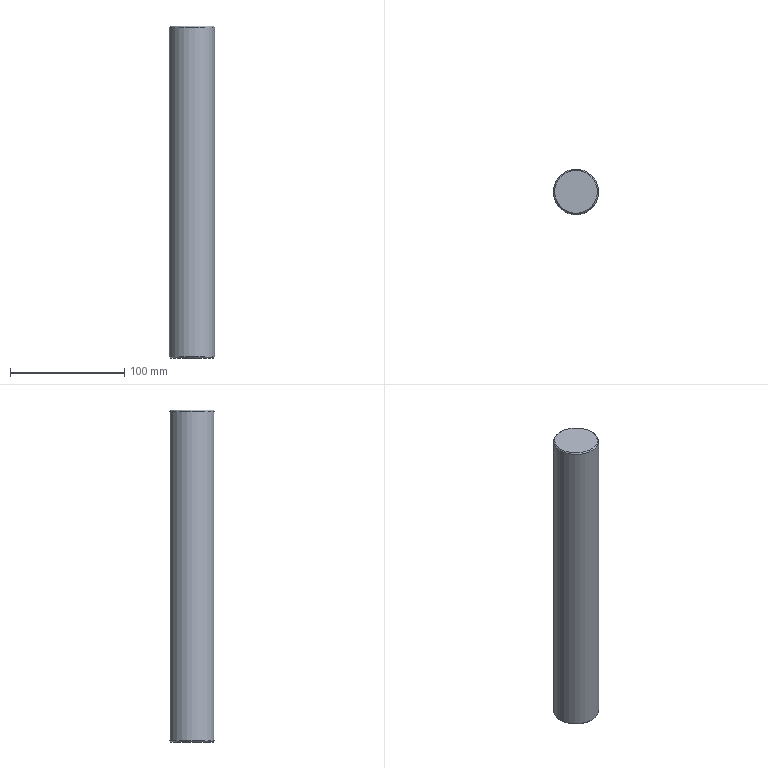Component | NX | STUD | 1 solid | 5 faces | box 39.47 x 39.47 x 290 mm | volume 354647 mm3 | plane 2 | cone 2 | cylinder 1 | commonest cylinder face diameters 39.467 x1
STEP:
#1=CARTESIAN_POINT('',(0.,0.,0.));
#2=DIRECTION('',(0.,0.,1.));
#3=DIRECTION('',(1.,0.,0.));
#4=AXIS2_PLACEMENT_3D('',#1,#2,#3);
#5=CARTESIAN_POINT('',(-41.267,165.,310.));
#6=VERTEX_POINT('',#5);
#7=CARTESIAN_POINT('',(-60.,165.,310.));
#8=DIRECTION('',(0.,0.,1.));
#9=DIRECTION('',(1.,0.,0.));
#10=AXIS2_PLACEMENT_3D('',#7,#8,#9);
#11=CIRCLE('',#10,18.733);
#12=CARTESIAN_POINT('',(-60.,165.,310.));
#13=DIRECTION('',(0.,0.,1.));
#14=DIRECTION('',(1.,0.,0.));
#15=AXIS2_PLACEMENT_3D('',#12,#13,#14);
#16=PLANE('',#15);
#17=CARTESIAN_POINT('',(0.,0.));
#18=DIRECTION('',(1.,0.));
#19=AXIS2_PLACEMENT_2D('',#17,#18);
#20=CIRCLE('',#19,18.733);
#21=(GEOMETRIC_REPRESENTATION_CONTEXT(2)PARAMETRIC_REPRESENTATION_CONTEXT()REPRESENTATION_CONTEXT('',''));
#22=DEFINITIONAL_REPRESENTATION('',(#20),#21);
#23=PCURVE('',#16,#22);
#24=CARTESIAN_POINT('',(-60.,165.,309.));
#25=DIRECTION('',(0.,0.,-1.));
#26=DIRECTION('',(-1.,0.,0.));
#27=AXIS2_PLACEMENT_3D('',#24,#25,#26);
#28=CONICAL_SURFACE('',#27,19.733,0.7854);
#29=CARTESIAN_POINT('',(9.425,-1.));
#30=DIRECTION('',(-1.,0.));
#31=VECTOR('',#30,1.);
#32=LINE('',#29,#31);
#33=(GEOMETRIC_REPRESENTATION_CONTEXT(2)PARAMETRIC_REPRESENTATION_CONTEXT()REPRESENTATION_CONTEXT('',''));
#34=DEFINITIONAL_REPRESENTATION('',(#32),#33);
#35=PCURVE('',#28,#34);
#36=SURFACE_CURVE('',#11,(#23,#35),.PCURVE_S1.);
#37=EDGE_CURVE('',#6,#6,#36,.T.);
#38=ORIENTED_EDGE('',*,*,#37,.T.);
#39=EDGE_LOOP('',(#38));
#40=FACE_BOUND('',#39,.T.);
#41=ADVANCED_FACE('',(#40),#16,.T.);
#42=CARTESIAN_POINT('',(-78.733,165.,20.));
#43=VERTEX_POINT('',#42);
#44=CARTESIAN_POINT('',(-60.,165.,20.));
#45=DIRECTION('',(0.,0.,-1.));
#46=DIRECTION('',(-1.,0.,0.));
#47=AXIS2_PLACEMENT_3D('',#44,#45,#46);
#48=CIRCLE('',#47,18.733);
#49=CARTESIAN_POINT('',(-60.,165.,20.));
#50=DIRECTION('',(0.,0.,-1.));
#51=DIRECTION('',(-1.,0.,0.));
#52=AXIS2_PLACEMENT_3D('',#49,#50,#51);
#53=PLANE('',#52);
#54=CARTESIAN_POINT('',(0.,0.));
#55=DIRECTION('',(1.,0.));
#56=AXIS2_PLACEMENT_2D('',#54,#55);
#57=CIRCLE('',#56,18.733);
#58=(GEOMETRIC_REPRESENTATION_CONTEXT(2)PARAMETRIC_REPRESENTATION_CONTEXT()REPRESENTATION_CONTEXT('',''));
#59=DEFINITIONAL_REPRESENTATION('',(#57),#58);
#60=PCURVE('',#53,#59);
#61=CARTESIAN_POINT('',(-60.,165.,21.));
#62=DIRECTION('',(0.,0.,1.));
#63=DIRECTION('',(1.,0.,0.));
#64=AXIS2_PLACEMENT_3D('',#61,#62,#63);
#65=CONICAL_SURFACE('',#64,19.733,0.7854);
#66=CARTESIAN_POINT('',(9.425,-1.));
#67=DIRECTION('',(-1.,0.));
#68=VECTOR('',#67,1.);
#69=LINE('',#66,#68);
#70=(GEOMETRIC_REPRESENTATION_CONTEXT(2)PARAMETRIC_REPRESENTATION_CONTEXT()REPRESENTATION_CONTEXT('',''));
#71=DEFINITIONAL_REPRESENTATION('',(#69),#70);
#72=PCURVE('',#65,#71);
#73=SURFACE_CURVE('',#48,(#60,#72),.PCURVE_S1.);
#74=EDGE_CURVE('',#43,#43,#73,.T.);
#75=ORIENTED_EDGE('',*,*,#74,.T.);
#76=EDGE_LOOP('',(#75));
#77=FACE_BOUND('',#76,.T.);
#78=ADVANCED_FACE('',(#77),#53,.T.);
#79=CARTESIAN_POINT('',(-40.267,165.,309.));
#80=VERTEX_POINT('',#79);
#81=CARTESIAN_POINT('',(-60.,165.,309.));
#82=DIRECTION('',(0.,0.,-1.));
#83=DIRECTION('',(1.,0.,0.));
#84=AXIS2_PLACEMENT_3D('',#81,#82,#83);
#85=CIRCLE('',#84,19.733);
#86=CARTESIAN_POINT('',(-60.,165.,20.));
#87=DIRECTION('',(0.,0.,1.));
#88=DIRECTION('',(1.,0.,0.));
#89=AXIS2_PLACEMENT_3D('',#86,#87,#88);
#90=CYLINDRICAL_SURFACE('',#89,19.733);
#91=CARTESIAN_POINT('',(6.283,289.));
#92=DIRECTION('',(-1.,0.));
#93=VECTOR('',#92,1.);
#94=LINE('',#91,#93);
#95=(GEOMETRIC_REPRESENTATION_CONTEXT(2)PARAMETRIC_REPRESENTATION_CONTEXT()REPRESENTATION_CONTEXT('',''));
#96=DEFINITIONAL_REPRESENTATION('',(#94),#95);
#97=PCURVE('',#90,#96);
#98=CARTESIAN_POINT('',(3.142,0.));
#99=DIRECTION('',(1.,0.));
#100=VECTOR('',#99,1.);
#101=LINE('',#98,#100);
#102=(GEOMETRIC_REPRESENTATION_CONTEXT(2)PARAMETRIC_REPRESENTATION_CONTEXT()REPRESENTATION_CONTEXT('',''));
#103=DEFINITIONAL_REPRESENTATION('',(#101),#102);
#104=PCURVE('',#28,#103);
#105=SURFACE_CURVE('',#85,(#97,#104),.PCURVE_S1.);
#106=EDGE_CURVE('',#80,#80,#105,.T.);
#107=ORIENTED_EDGE('',*,*,#106,.T.);
#108=CARTESIAN_POINT('',(-40.267,165.,21.));
#109=VERTEX_POINT('',#108);
#110=CARTESIAN_POINT('',(-40.267,165.,21.));
#111=CARTESIAN_POINT('',(-40.267,165.,309.));
#112=B_SPLINE_CURVE_WITH_KNOTS('',1,(#110,#111),.UNSPECIFIED.,.F.,.F.,(2,2),(1.,289.),.PIECEWISE_BEZIER_KNOTS.);
#113=CARTESIAN_POINT('',(0.,0.));
#114=DIRECTION('',(0.,1.));
#115=VECTOR('',#114,1.);
#116=LINE('',#113,#115);
#117=(GEOMETRIC_REPRESENTATION_CONTEXT(2)PARAMETRIC_REPRESENTATION_CONTEXT()REPRESENTATION_CONTEXT('',''));
#118=DEFINITIONAL_REPRESENTATION('',(#116),#117);
#119=PCURVE('',#90,#118);
#120=CARTESIAN_POINT('',(6.283,0.));
#121=DIRECTION('',(0.,1.));
#122=VECTOR('',#121,1.);
#123=LINE('',#120,#122);
#124=(GEOMETRIC_REPRESENTATION_CONTEXT(2)PARAMETRIC_REPRESENTATION_CONTEXT()REPRESENTATION_CONTEXT('',''));
#125=DEFINITIONAL_REPRESENTATION('',(#123),#124);
#126=PCURVE('',#90,#125);
#127=SEAM_CURVE('',#112,(#119,#126),.PCURVE_S1.);
#128=EDGE_CURVE('',#109,#80,#127,.T.);
#129=ORIENTED_EDGE('',*,*,#128,.F.);
#130=CARTESIAN_POINT('',(-79.733,165.,21.));
#131=VERTEX_POINT('',#130);
#132=CARTESIAN_POINT('',(-60.,165.,21.));
#133=DIRECTION('',(0.,0.,1.));
#134=DIRECTION('',(-1.,0.,0.));
#135=AXIS2_PLACEMENT_3D('',#132,#133,#134);
#136=CIRCLE('',#135,19.733);
#137=CARTESIAN_POINT('',(-3.142,1.));
#138=DIRECTION('',(1.,0.));
#139=VECTOR('',#138,1.);
#140=LINE('',#137,#139);
#141=(GEOMETRIC_REPRESENTATION_CONTEXT(2)PARAMETRIC_REPRESENTATION_CONTEXT()REPRESENTATION_CONTEXT('',''));
#142=DEFINITIONAL_REPRESENTATION('',(#140),#141);
#143=PCURVE('',#90,#142);
#144=CARTESIAN_POINT('',(3.142,0.));
#145=DIRECTION('',(1.,0.));
#146=VECTOR('',#145,1.);
#147=LINE('',#144,#146);
#148=(GEOMETRIC_REPRESENTATION_CONTEXT(2)PARAMETRIC_REPRESENTATION_CONTEXT()REPRESENTATION_CONTEXT('',''));
#149=DEFINITIONAL_REPRESENTATION('',(#147),#148);
#150=PCURVE('',#65,#149);
#151=SURFACE_CURVE('',#136,(#143,#150),.PCURVE_S1.);
#152=EDGE_CURVE('',#109,#131,#151,.T.);
#153=ORIENTED_EDGE('',*,*,#152,.T.);
#154=CARTESIAN_POINT('',(-60.,165.,21.));
#155=DIRECTION('',(0.,0.,1.));
#156=DIRECTION('',(-1.,0.,0.));
#157=AXIS2_PLACEMENT_3D('',#154,#155,#156);
#158=CIRCLE('',#157,19.733);
#159=CARTESIAN_POINT('',(3.142,1.));
#160=DIRECTION('',(1.,0.));
#161=VECTOR('',#160,1.);
#162=LINE('',#159,#161);
#163=(GEOMETRIC_REPRESENTATION_CONTEXT(2)PARAMETRIC_REPRESENTATION_CONTEXT()REPRESENTATION_CONTEXT('',''));
#164=DEFINITIONAL_REPRESENTATION('',(#162),#163);
#165=PCURVE('',#90,#164);
#166=CARTESIAN_POINT('',(3.142,0.));
#167=DIRECTION('',(1.,0.));
#168=VECTOR('',#167,1.);
#169=LINE('',#166,#168);
#170=(GEOMETRIC_REPRESENTATION_CONTEXT(2)PARAMETRIC_REPRESENTATION_CONTEXT()REPRESENTATION_CONTEXT('',''));
#171=DEFINITIONAL_REPRESENTATION('',(#169),#170);
#172=PCURVE('',#65,#171);
#173=SURFACE_CURVE('',#158,(#165,#172),.PCURVE_S1.);
#174=EDGE_CURVE('',#131,#109,#173,.T.);
#175=ORIENTED_EDGE('',*,*,#174,.T.);
#176=ORIENTED_EDGE('',*,*,#128,.T.);
#177=EDGE_LOOP('',(#107,#129,#153,#175,#176));
#178=FACE_BOUND('',#177,.T.);
#179=ADVANCED_FACE('',(#178),#90,.T.);
#180=ORIENTED_EDGE('',*,*,#74,.F.);
#181=CARTESIAN_POINT('',(-78.733,165.,20.));
#182=CARTESIAN_POINT('',(-79.733,165.,21.));
#183=B_SPLINE_CURVE_WITH_KNOTS('',1,(#181,#182),.UNSPECIFIED.,.F.,.F.,(2,2),(-1.414,0.),.PIECEWISE_BEZIER_KNOTS.);
#184=CARTESIAN_POINT('',(9.425,0.));
#185=DIRECTION('',(0.,1.));
#186=VECTOR('',#185,1.);
#187=LINE('',#184,#186);
#188=(GEOMETRIC_REPRESENTATION_CONTEXT(2)PARAMETRIC_REPRESENTATION_CONTEXT()REPRESENTATION_CONTEXT('',''));
#189=DEFINITIONAL_REPRESENTATION('',(#187),#188);
#190=PCURVE('',#65,#189);
#191=CARTESIAN_POINT('',(3.142,0.));
#192=DIRECTION('',(0.,1.));
#193=VECTOR('',#192,1.);
#194=LINE('',#191,#193);
#195=(GEOMETRIC_REPRESENTATION_CONTEXT(2)PARAMETRIC_REPRESENTATION_CONTEXT()REPRESENTATION_CONTEXT('',''));
#196=DEFINITIONAL_REPRESENTATION('',(#194),#195);
#197=PCURVE('',#65,#196);
#198=SEAM_CURVE('',#183,(#190,#197),.PCURVE_S1.);
#199=EDGE_CURVE('',#43,#131,#198,.T.);
#200=ORIENTED_EDGE('',*,*,#199,.T.);
#201=ORIENTED_EDGE('',*,*,#152,.F.);
#202=ORIENTED_EDGE('',*,*,#174,.F.);
#203=ORIENTED_EDGE('',*,*,#199,.F.);
#204=EDGE_LOOP('',(#180,#200,#201,#202,#203));
#205=FACE_BOUND('',#204,.T.);
#206=ADVANCED_FACE('',(#205),#65,.T.);
#207=ORIENTED_EDGE('',*,*,#37,.F.);
#208=CARTESIAN_POINT('',(-41.267,165.,310.));
#209=CARTESIAN_POINT('',(-40.267,165.,309.));
#210=B_SPLINE_CURVE_WITH_KNOTS('',1,(#208,#209),.UNSPECIFIED.,.F.,.F.,(2,2),(-1.414,0.),.PIECEWISE_BEZIER_KNOTS.);
#211=CARTESIAN_POINT('',(9.425,0.));
#212=DIRECTION('',(0.,1.));
#213=VECTOR('',#212,1.);
#214=LINE('',#211,#213);
#215=(GEOMETRIC_REPRESENTATION_CONTEXT(2)PARAMETRIC_REPRESENTATION_CONTEXT()REPRESENTATION_CONTEXT('',''));
#216=DEFINITIONAL_REPRESENTATION('',(#214),#215);
#217=PCURVE('',#28,#216);
#218=CARTESIAN_POINT('',(3.142,0.));
#219=DIRECTION('',(0.,1.));
#220=VECTOR('',#219,1.);
#221=LINE('',#218,#220);
#222=(GEOMETRIC_REPRESENTATION_CONTEXT(2)PARAMETRIC_REPRESENTATION_CONTEXT()REPRESENTATION_CONTEXT('',''));
#223=DEFINITIONAL_REPRESENTATION('',(#221),#222);
#224=PCURVE('',#28,#223);
#225=SEAM_CURVE('',#210,(#217,#224),.PCURVE_S1.);
#226=EDGE_CURVE('',#6,#80,#225,.T.);
#227=ORIENTED_EDGE('',*,*,#226,.T.);
#228=ORIENTED_EDGE('',*,*,#106,.F.);
#229=ORIENTED_EDGE('',*,*,#226,.F.);
#230=EDGE_LOOP('',(#207,#227,#228,#229));
#231=FACE_BOUND('',#230,.T.);
#232=ADVANCED_FACE('',(#231),#28,.T.);
#233=CLOSED_SHELL('',(#41,#78,#179,#206,#232));
#234=MANIFOLD_SOLID_BREP('',#233);
#235=(LENGTH_UNIT()NAMED_UNIT(*)SI_UNIT(.MILLI.,.METRE.));
#236=UNCERTAINTY_MEASURE_WITH_UNIT(LENGTH_MEASURE(0.00001),#235,'','');
#237=(NAMED_UNIT(*)PLANE_ANGLE_UNIT()SI_UNIT($,.RADIAN.));
#238=(NAMED_UNIT(*)SI_UNIT($,.STERADIAN.)SOLID_ANGLE_UNIT());
#239=(GEOMETRIC_REPRESENTATION_CONTEXT(3)GLOBAL_UNCERTAINTY_ASSIGNED_CONTEXT((#236))GLOBAL_UNIT_ASSIGNED_CONTEXT((#235,#237,#238))REPRESENTATION_CONTEXT('',''));
#240=ADVANCED_BREP_SHAPE_REPRESENTATION('',(#4,#234),#239);